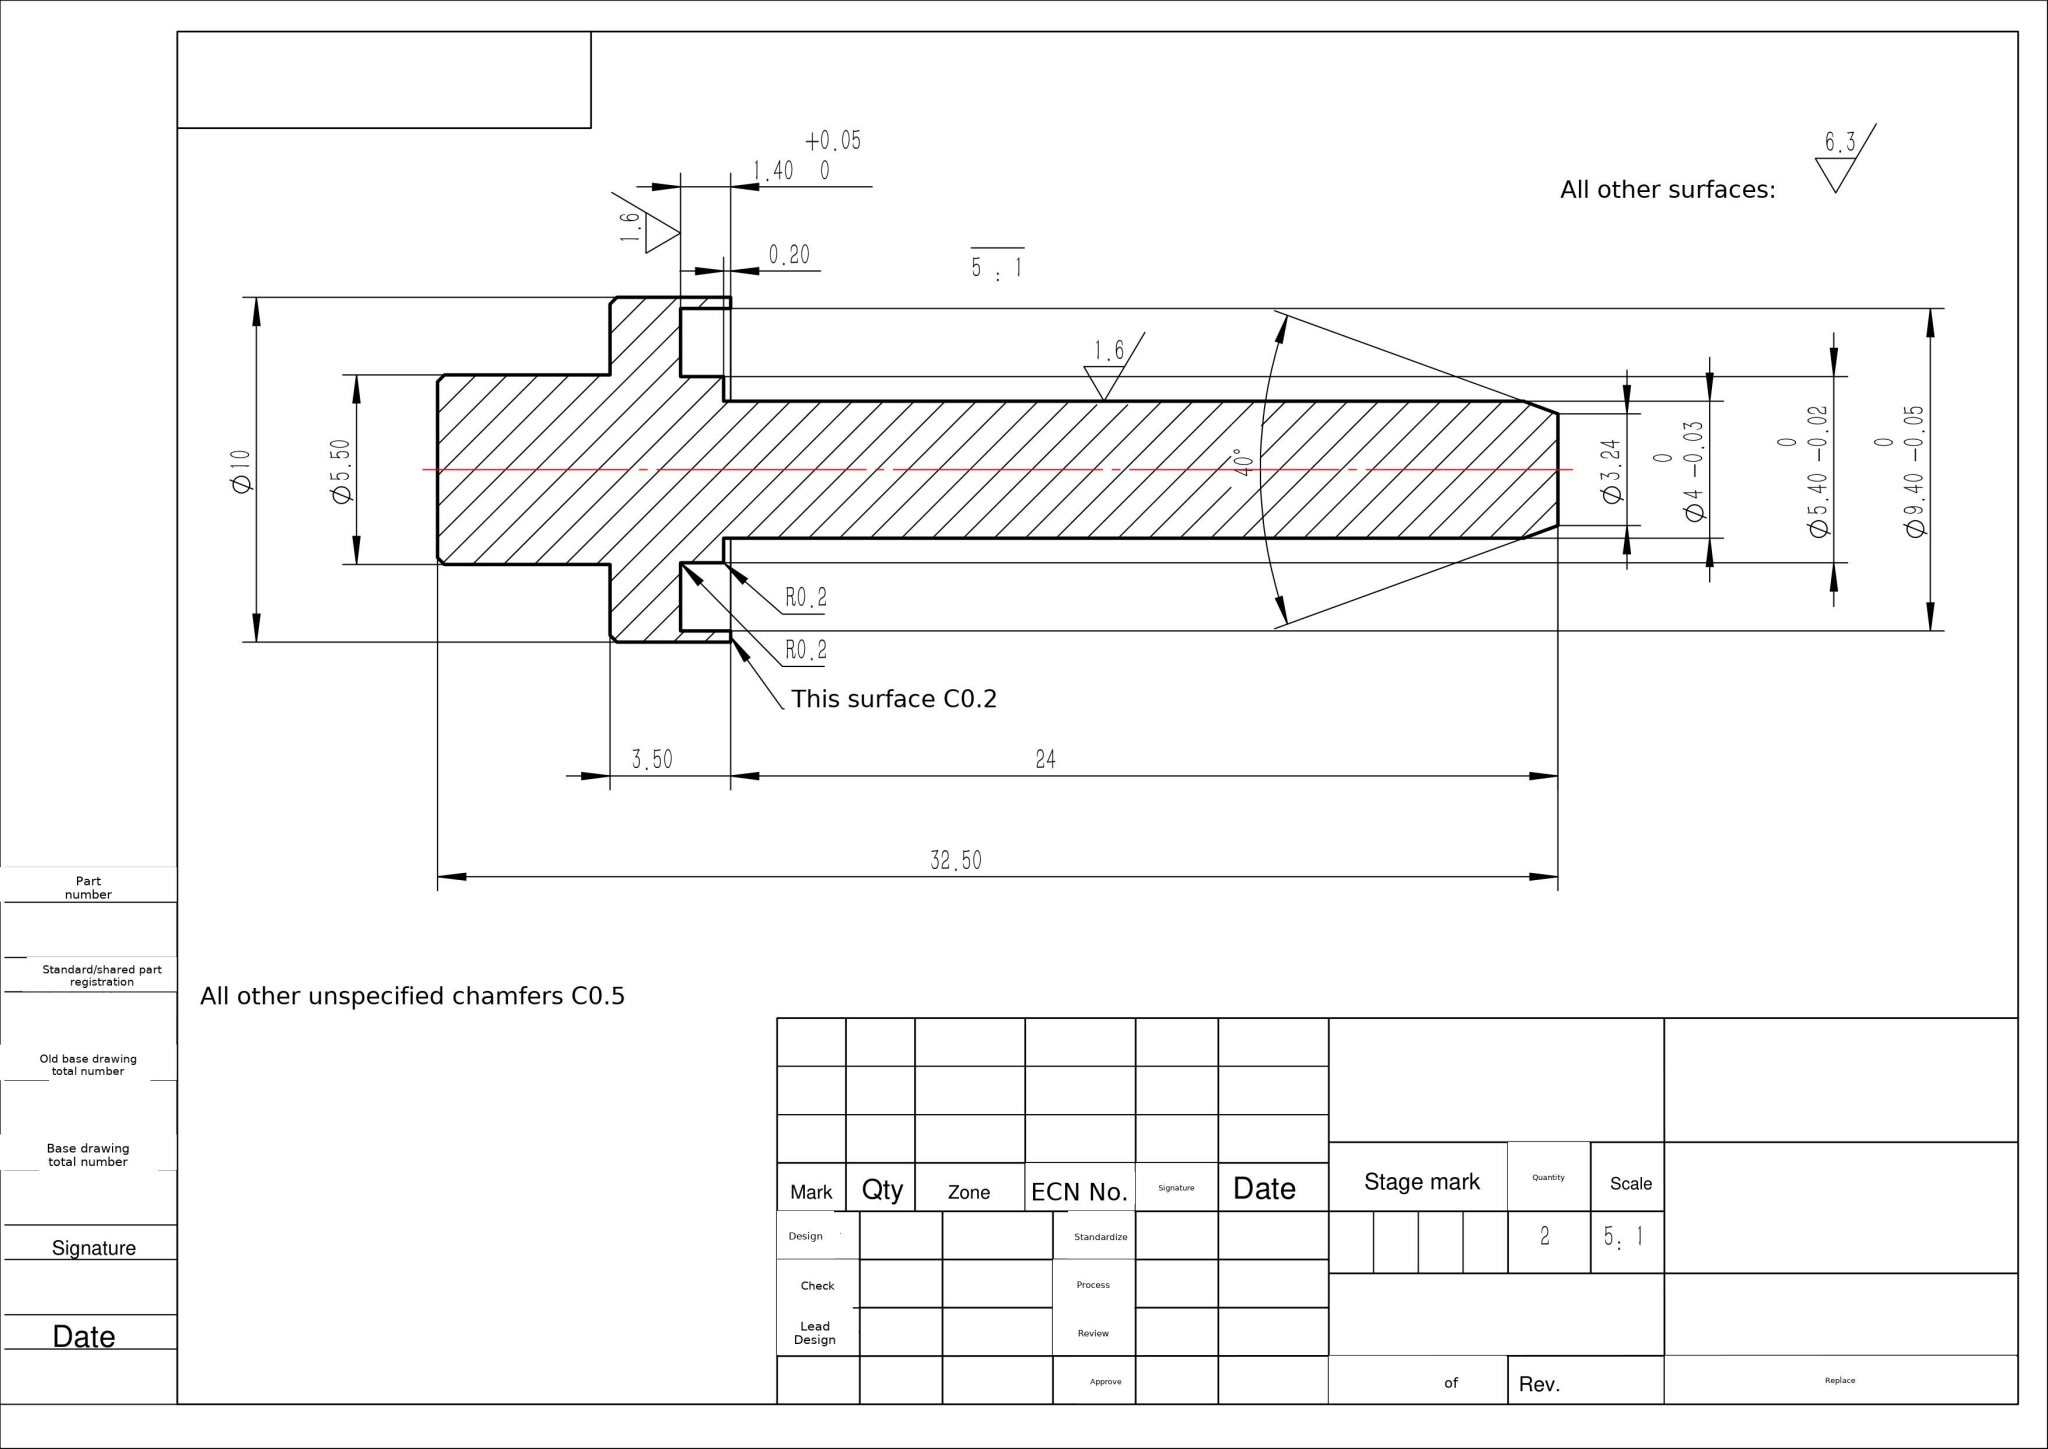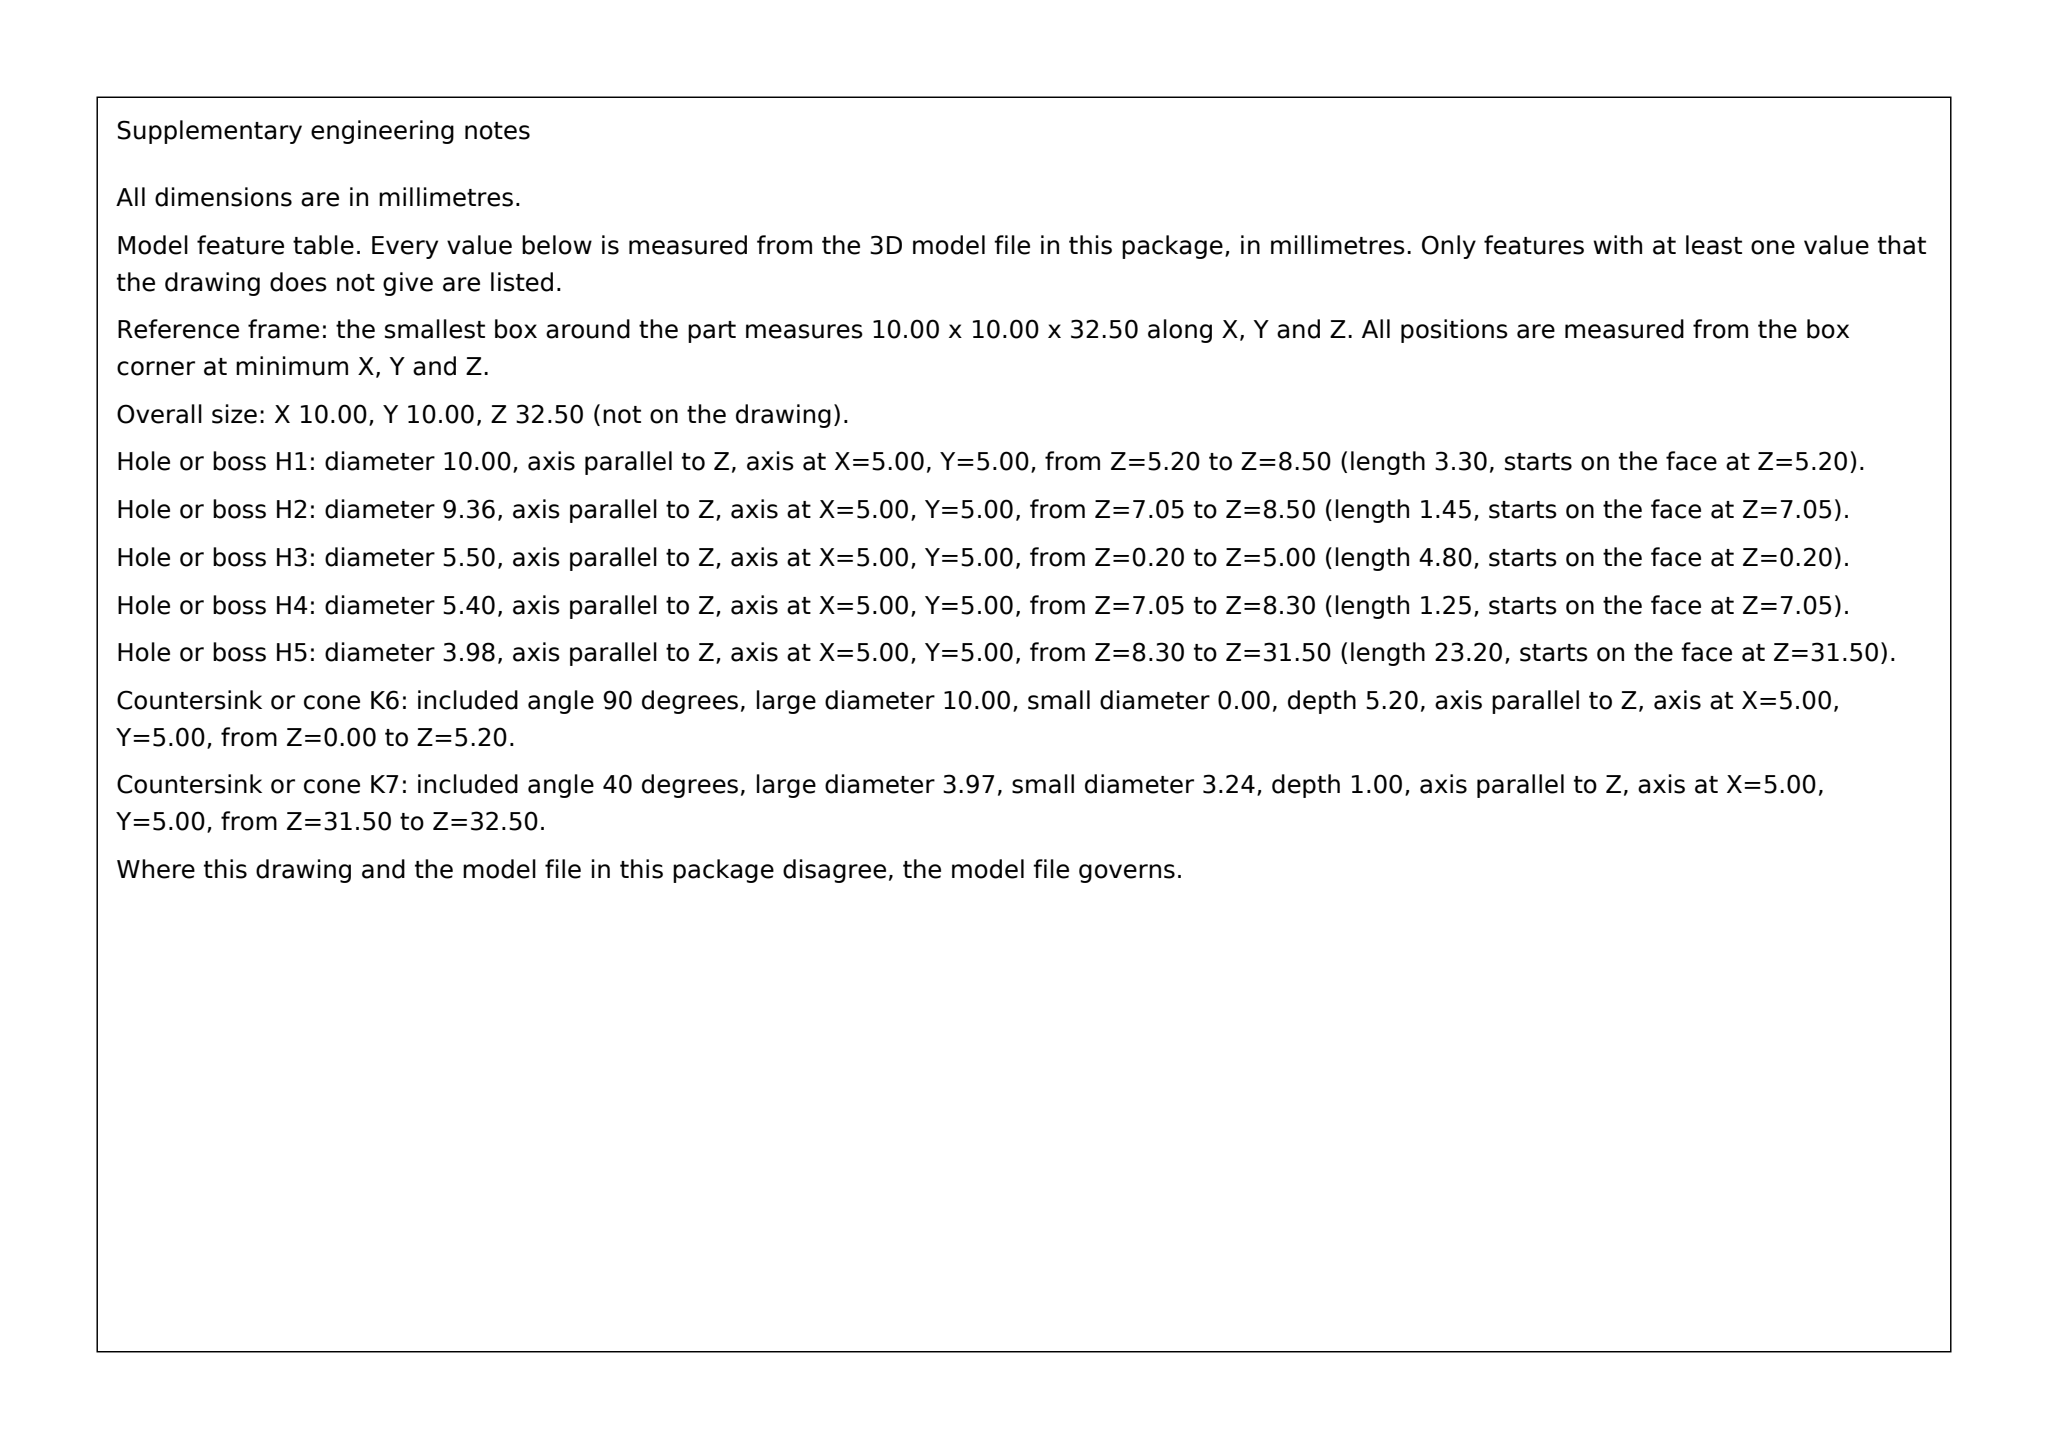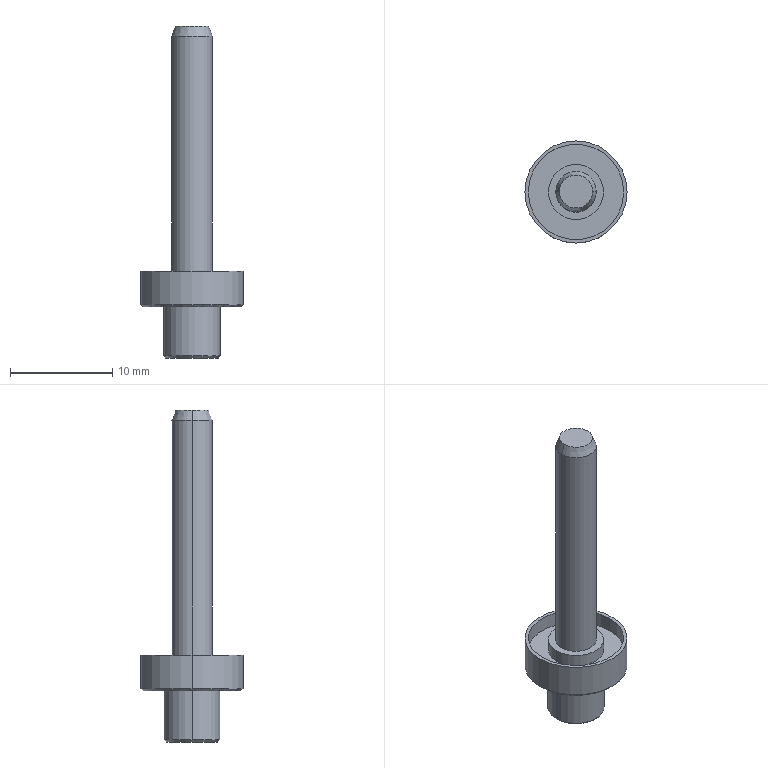Part | SolidWorks | mm | 1 solid | 22 faces | box 10 x 10 x 32.5 mm | volume 619 mm3 | cylinder 10 | cone 6 | plane 6 | commonest cylinder face diameters 3.97 x2 5.4 x2 9.35 x2 10 x2 5.5 x2
build123d program:
from build123d import *

# Parameters (mm, degrees)
CHAMFER1_SIZE  = 0.2
CHAMFER2_SIZE  = 1
CHAMFER2_SIZE2 = 0.364


with BuildPart() as part:
    # Sketch1 → Revolve1 (revolve)
    with BuildSketch(Plane(origin=(0, 0, 0), x_dir=(0, 0, -1), z_dir=(1, 0, 0)), mode=Mode.PRIVATE) as revolve1_sk:
        Polygon((32.5, 0), (32.5, 2.75), (27.5, 2.75), (27.5, 5), (24, 5), (24, 4.675), (25.45, 4.675), (25.45, 2.7), (24.2, 2.7), (24.2, 1.985), (0, 1.985), (0, 0), align=None)
    revolve(revolve1_sk.sketch.rotate(Axis((0, 0, 0), (0, 0, -1)), 90), axis=Axis((0, 0, 0), (0, 0, -1)))

    # Chamfer1
    chamfer1_edges = [part.edges().sort_by_distance(p)[0] for p in [
        (-5, 0, -27.5),
        (-2.75, 0, -32.5),
    ]]
    chamfer(chamfer1_edges, length=CHAMFER1_SIZE)

    # Chamfer2
    chamfer2_edges = [part.edges().sort_by_distance(p)[0] for p in [
        (-1.985, 0, 0),
    ]]
    chamfer2_side = [part.faces().sort_by_distance(p)[0] for p in [
        (-1.985, 0, -12.1),
    ]]
    chamfer(chamfer2_edges, length=CHAMFER2_SIZE, length2=CHAMFER2_SIZE2, reference=chamfer2_side[0])


solid = part.part
STEP:
#1=CARTESIAN_POINT('',(1.621,0.,-0.));
#2=VERTEX_POINT('',#1);
#3=CARTESIAN_POINT('',(-1.621,0.,-0.));
#4=VERTEX_POINT('',#3);
#5=CARTESIAN_POINT('',(0.,0.,0.));
#6=DIRECTION('',(0.,0.,1.));
#7=DIRECTION('',(-1.,0.,-0.));
#8=AXIS2_PLACEMENT_3D('',#5,#6,#7);
#9=CIRCLE('',#8,1.621);
#10=EDGE_CURVE('',#2,#4,#9,.T.);
#11=ORIENTED_EDGE('',*,*,#10,.F.);
#12=CARTESIAN_POINT('',(1.985,-0.,-1.));
#13=VERTEX_POINT('',#12);
#14=CARTESIAN_POINT('',(1.621,0.,0.));
#15=DIRECTION('',(0.342,0.,-0.9397));
#16=VECTOR('',#15,1000.);
#17=LINE('',#14,#16);
#18=EDGE_CURVE('',#2,#13,#17,.T.);
#19=ORIENTED_EDGE('',*,*,#18,.T.);
#20=CARTESIAN_POINT('',(-1.985,0.,-1.));
#21=VERTEX_POINT('',#20);
#22=CARTESIAN_POINT('',(0.,0.,-1.));
#23=DIRECTION('',(-0.,-0.,-1.));
#24=DIRECTION('',(-1.,0.,0.));
#25=AXIS2_PLACEMENT_3D('',#22,#23,#24);
#26=CIRCLE('',#25,1.985);
#27=EDGE_CURVE('',#21,#13,#26,.T.);
#28=ORIENTED_EDGE('',*,*,#27,.F.);
#29=CARTESIAN_POINT('',(-1.621,0.,-0.));
#30=DIRECTION('',(-0.342,0.,-0.9397));
#31=VECTOR('',#30,1000.);
#32=LINE('',#29,#31);
#33=EDGE_CURVE('',#4,#21,#32,.T.);
#34=ORIENTED_EDGE('',*,*,#33,.F.);
#35=EDGE_LOOP('',(#11,#19,#28,#34));
#36=FACE_OUTER_BOUND('',#35,.T.);
#37=CARTESIAN_POINT('',(0.,0.,0.));
#38=DIRECTION('',(-0.,-0.,-1.));
#39=DIRECTION('',(-1.,0.,-0.));
#40=AXIS2_PLACEMENT_3D('',#37,#38,#39);
#41=CONICAL_SURFACE('',#40,1.621,0.3491);
#42=ADVANCED_FACE('',(#36),#41,.T.);
#43=CARTESIAN_POINT('',(-2.55,0.,-32.5));
#44=VERTEX_POINT('',#43);
#45=CARTESIAN_POINT('',(2.55,0.,-32.5));
#46=VERTEX_POINT('',#45);
#47=CARTESIAN_POINT('',(0.,0.,-32.5));
#48=DIRECTION('',(-0.,-0.,-1.));
#49=DIRECTION('',(1.,-0.,0.));
#50=AXIS2_PLACEMENT_3D('',#47,#48,#49);
#51=CIRCLE('',#50,2.55);
#52=EDGE_CURVE('',#44,#46,#51,.T.);
#53=ORIENTED_EDGE('',*,*,#52,.F.);
#54=CARTESIAN_POINT('',(-2.75,0.,-32.3));
#55=VERTEX_POINT('',#54);
#56=CARTESIAN_POINT('',(-2.75,0.,-32.3));
#57=DIRECTION('',(-0.7071,0.,0.7071));
#58=VECTOR('',#57,1000.);
#59=LINE('',#56,#58);
#60=EDGE_CURVE('',#44,#55,#59,.T.);
#61=ORIENTED_EDGE('',*,*,#60,.T.);
#62=CARTESIAN_POINT('',(2.75,0.,-32.3));
#63=VERTEX_POINT('',#62);
#64=CARTESIAN_POINT('',(0.,0.,-32.3));
#65=DIRECTION('',(0.,0.,1.));
#66=DIRECTION('',(1.,-0.,0.));
#67=AXIS2_PLACEMENT_3D('',#64,#65,#66);
#68=CIRCLE('',#67,2.75);
#69=EDGE_CURVE('',#63,#55,#68,.T.);
#70=ORIENTED_EDGE('',*,*,#69,.F.);
#71=CARTESIAN_POINT('',(2.75,0.,-32.3));
#72=DIRECTION('',(0.7071,-0.,0.7071));
#73=VECTOR('',#72,1000.);
#74=LINE('',#71,#73);
#75=EDGE_CURVE('',#46,#63,#74,.T.);
#76=ORIENTED_EDGE('',*,*,#75,.F.);
#77=EDGE_LOOP('',(#53,#61,#70,#76));
#78=FACE_OUTER_BOUND('',#77,.T.);
#79=CARTESIAN_POINT('',(0.,0.,-32.3));
#80=DIRECTION('',(0.,0.,1.));
#81=DIRECTION('',(1.,-0.,0.));
#82=AXIS2_PLACEMENT_3D('',#79,#80,#81);
#83=CONICAL_SURFACE('',#82,2.75,0.7854);
#84=ADVANCED_FACE('',(#78),#83,.T.);
#85=CARTESIAN_POINT('',(-4.8,0.,-27.5));
#86=VERTEX_POINT('',#85);
#87=CARTESIAN_POINT('',(4.8,0.,-27.5));
#88=VERTEX_POINT('',#87);
#89=CARTESIAN_POINT('',(0.,0.,-27.5));
#90=DIRECTION('',(-0.,-0.,-1.));
#91=DIRECTION('',(1.,-0.,0.));
#92=AXIS2_PLACEMENT_3D('',#89,#90,#91);
#93=CIRCLE('',#92,4.8);
#94=EDGE_CURVE('',#86,#88,#93,.T.);
#95=ORIENTED_EDGE('',*,*,#94,.F.);
#96=CARTESIAN_POINT('',(-5.,0.,-27.3));
#97=VERTEX_POINT('',#96);
#98=CARTESIAN_POINT('',(-5.,0.,-27.3));
#99=DIRECTION('',(-0.7071,0.,0.7071));
#100=VECTOR('',#99,1000.);
#101=LINE('',#98,#100);
#102=EDGE_CURVE('',#86,#97,#101,.T.);
#103=ORIENTED_EDGE('',*,*,#102,.T.);
#104=CARTESIAN_POINT('',(5.,0.,-27.3));
#105=VERTEX_POINT('',#104);
#106=CARTESIAN_POINT('',(0.,0.,-27.3));
#107=DIRECTION('',(0.,0.,1.));
#108=DIRECTION('',(1.,-0.,0.));
#109=AXIS2_PLACEMENT_3D('',#106,#107,#108);
#110=CIRCLE('',#109,5.);
#111=EDGE_CURVE('',#105,#97,#110,.T.);
#112=ORIENTED_EDGE('',*,*,#111,.F.);
#113=CARTESIAN_POINT('',(5.,0.,-27.3));
#114=DIRECTION('',(0.7071,-0.,0.7071));
#115=VECTOR('',#114,1000.);
#116=LINE('',#113,#115);
#117=EDGE_CURVE('',#88,#105,#116,.T.);
#118=ORIENTED_EDGE('',*,*,#117,.F.);
#119=EDGE_LOOP('',(#95,#103,#112,#118));
#120=FACE_OUTER_BOUND('',#119,.T.);
#121=CARTESIAN_POINT('',(0.,0.,-27.3));
#122=DIRECTION('',(0.,0.,1.));
#123=DIRECTION('',(1.,-0.,0.));
#124=AXIS2_PLACEMENT_3D('',#121,#122,#123);
#125=CONICAL_SURFACE('',#124,5.,0.7854);
#126=ADVANCED_FACE('',(#120),#125,.T.);
#127=CARTESIAN_POINT('',(1.985,0.,-24.2));
#128=VERTEX_POINT('',#127);
#129=CARTESIAN_POINT('',(-1.985,0.,-24.2));
#130=VERTEX_POINT('',#129);
#131=CARTESIAN_POINT('',(0.,0.,-24.2));
#132=DIRECTION('',(0.,0.,1.));
#133=DIRECTION('',(1.,-0.,0.));
#134=AXIS2_PLACEMENT_3D('',#131,#132,#133);
#135=CIRCLE('',#134,1.985);
#136=EDGE_CURVE('',#128,#130,#135,.T.);
#137=ORIENTED_EDGE('',*,*,#136,.T.);
#138=CARTESIAN_POINT('',(-1.985,0.,-0.));
#139=DIRECTION('',(0.,0.,1.));
#140=VECTOR('',#139,1000.);
#141=LINE('',#138,#140);
#142=EDGE_CURVE('',#130,#21,#141,.T.);
#143=ORIENTED_EDGE('',*,*,#142,.T.);
#144=ORIENTED_EDGE('',*,*,#27,.T.);
#145=CARTESIAN_POINT('',(1.985,-0.,0.));
#146=DIRECTION('',(0.,0.,1.));
#147=VECTOR('',#146,1000.);
#148=LINE('',#145,#147);
#149=EDGE_CURVE('',#128,#13,#148,.T.);
#150=ORIENTED_EDGE('',*,*,#149,.F.);
#151=EDGE_LOOP('',(#137,#143,#144,#150));
#152=FACE_OUTER_BOUND('',#151,.T.);
#153=CARTESIAN_POINT('',(0.,0.,0.));
#154=DIRECTION('',(0.,0.,1.));
#155=DIRECTION('',(1.,-0.,0.));
#156=AXIS2_PLACEMENT_3D('',#153,#154,#155);
#157=CYLINDRICAL_SURFACE('',#156,1.985);
#158=ADVANCED_FACE('',(#152),#157,.T.);
#159=CARTESIAN_POINT('',(2.7,0.,-25.45));
#160=VERTEX_POINT('',#159);
#161=CARTESIAN_POINT('',(-2.7,0.,-25.45));
#162=VERTEX_POINT('',#161);
#163=CARTESIAN_POINT('',(0.,0.,-25.45));
#164=DIRECTION('',(0.,0.,1.));
#165=DIRECTION('',(1.,-0.,0.));
#166=AXIS2_PLACEMENT_3D('',#163,#164,#165);
#167=CIRCLE('',#166,2.7);
#168=EDGE_CURVE('',#160,#162,#167,.T.);
#169=ORIENTED_EDGE('',*,*,#168,.T.);
#170=CARTESIAN_POINT('',(-2.7,0.,-24.2));
#171=VERTEX_POINT('',#170);
#172=CARTESIAN_POINT('',(-2.7,0.,-0.));
#173=DIRECTION('',(0.,0.,1.));
#174=VECTOR('',#173,1000.);
#175=LINE('',#172,#174);
#176=EDGE_CURVE('',#162,#171,#175,.T.);
#177=ORIENTED_EDGE('',*,*,#176,.T.);
#178=CARTESIAN_POINT('',(2.7,0.,-24.2));
#179=VERTEX_POINT('',#178);
#180=CARTESIAN_POINT('',(0.,0.,-24.2));
#181=DIRECTION('',(0.,0.,1.));
#182=DIRECTION('',(1.,-0.,0.));
#183=AXIS2_PLACEMENT_3D('',#180,#181,#182);
#184=CIRCLE('',#183,2.7);
#185=EDGE_CURVE('',#179,#171,#184,.T.);
#186=ORIENTED_EDGE('',*,*,#185,.F.);
#187=CARTESIAN_POINT('',(2.7,-0.,0.));
#188=DIRECTION('',(0.,0.,1.));
#189=VECTOR('',#188,1000.);
#190=LINE('',#187,#189);
#191=EDGE_CURVE('',#160,#179,#190,.T.);
#192=ORIENTED_EDGE('',*,*,#191,.F.);
#193=EDGE_LOOP('',(#169,#177,#186,#192));
#194=FACE_OUTER_BOUND('',#193,.T.);
#195=CARTESIAN_POINT('',(0.,0.,0.));
#196=DIRECTION('',(0.,0.,1.));
#197=DIRECTION('',(1.,-0.,0.));
#198=AXIS2_PLACEMENT_3D('',#195,#196,#197);
#199=CYLINDRICAL_SURFACE('',#198,2.7);
#200=ADVANCED_FACE('',(#194),#199,.T.);
#201=CARTESIAN_POINT('',(-4.675,0.,-25.45));
#202=VERTEX_POINT('',#201);
#203=CARTESIAN_POINT('',(4.675,0.,-25.45));
#204=VERTEX_POINT('',#203);
#205=CARTESIAN_POINT('',(0.,0.,-25.45));
#206=DIRECTION('',(0.,0.,1.));
#207=DIRECTION('',(1.,-0.,0.));
#208=AXIS2_PLACEMENT_3D('',#205,#206,#207);
#209=CIRCLE('',#208,4.675);
#210=EDGE_CURVE('',#202,#204,#209,.T.);
#211=ORIENTED_EDGE('',*,*,#210,.F.);
#212=CARTESIAN_POINT('',(-4.675,0.,-24.));
#213=VERTEX_POINT('',#212);
#214=CARTESIAN_POINT('',(-4.675,0.,-0.));
#215=DIRECTION('',(0.,0.,1.));
#216=VECTOR('',#215,1000.);
#217=LINE('',#214,#216);
#218=EDGE_CURVE('',#202,#213,#217,.T.);
#219=ORIENTED_EDGE('',*,*,#218,.T.);
#220=CARTESIAN_POINT('',(4.675,0.,-24.));
#221=VERTEX_POINT('',#220);
#222=CARTESIAN_POINT('',(0.,0.,-24.));
#223=DIRECTION('',(0.,0.,1.));
#224=DIRECTION('',(1.,-0.,0.));
#225=AXIS2_PLACEMENT_3D('',#222,#223,#224);
#226=CIRCLE('',#225,4.675);
#227=EDGE_CURVE('',#213,#221,#226,.T.);
#228=ORIENTED_EDGE('',*,*,#227,.T.);
#229=CARTESIAN_POINT('',(4.675,-0.,0.));
#230=DIRECTION('',(0.,0.,1.));
#231=VECTOR('',#230,1000.);
#232=LINE('',#229,#231);
#233=EDGE_CURVE('',#204,#221,#232,.T.);
#234=ORIENTED_EDGE('',*,*,#233,.F.);
#235=EDGE_LOOP('',(#211,#219,#228,#234));
#236=FACE_OUTER_BOUND('',#235,.T.);
#237=CARTESIAN_POINT('',(0.,0.,0.));
#238=DIRECTION('',(0.,0.,1.));
#239=DIRECTION('',(1.,-0.,0.));
#240=AXIS2_PLACEMENT_3D('',#237,#238,#239);
#241=CYLINDRICAL_SURFACE('',#240,4.675);
#242=ADVANCED_FACE('',(#236),#241,.F.);
#243=ORIENTED_EDGE('',*,*,#111,.T.);
#244=CARTESIAN_POINT('',(-5.,0.,-24.));
#245=VERTEX_POINT('',#244);
#246=CARTESIAN_POINT('',(-5.,0.,-0.));
#247=DIRECTION('',(0.,0.,1.));
#248=VECTOR('',#247,1000.);
#249=LINE('',#246,#248);
#250=EDGE_CURVE('',#97,#245,#249,.T.);
#251=ORIENTED_EDGE('',*,*,#250,.T.);
#252=CARTESIAN_POINT('',(5.,0.,-24.));
#253=VERTEX_POINT('',#252);
#254=CARTESIAN_POINT('',(0.,0.,-24.));
#255=DIRECTION('',(0.,0.,1.));
#256=DIRECTION('',(1.,-0.,0.));
#257=AXIS2_PLACEMENT_3D('',#254,#255,#256);
#258=CIRCLE('',#257,5.);
#259=EDGE_CURVE('',#253,#245,#258,.T.);
#260=ORIENTED_EDGE('',*,*,#259,.F.);
#261=CARTESIAN_POINT('',(5.,-0.,0.));
#262=DIRECTION('',(0.,0.,1.));
#263=VECTOR('',#262,1000.);
#264=LINE('',#261,#263);
#265=EDGE_CURVE('',#105,#253,#264,.T.);
#266=ORIENTED_EDGE('',*,*,#265,.F.);
#267=EDGE_LOOP('',(#243,#251,#260,#266));
#268=FACE_OUTER_BOUND('',#267,.T.);
#269=CARTESIAN_POINT('',(0.,0.,0.));
#270=DIRECTION('',(0.,0.,1.));
#271=DIRECTION('',(1.,-0.,0.));
#272=AXIS2_PLACEMENT_3D('',#269,#270,#271);
#273=CYLINDRICAL_SURFACE('',#272,5.);
#274=ADVANCED_FACE('',(#268),#273,.T.);
#275=ORIENTED_EDGE('',*,*,#69,.T.);
#276=CARTESIAN_POINT('',(-2.75,0.,-27.5));
#277=VERTEX_POINT('',#276);
#278=CARTESIAN_POINT('',(-2.75,0.,-0.));
#279=DIRECTION('',(0.,0.,1.));
#280=VECTOR('',#279,1000.);
#281=LINE('',#278,#280);
#282=EDGE_CURVE('',#55,#277,#281,.T.);
#283=ORIENTED_EDGE('',*,*,#282,.T.);
#284=CARTESIAN_POINT('',(2.75,0.,-27.5));
#285=VERTEX_POINT('',#284);
#286=CARTESIAN_POINT('',(0.,0.,-27.5));
#287=DIRECTION('',(0.,0.,1.));
#288=DIRECTION('',(1.,-0.,0.));
#289=AXIS2_PLACEMENT_3D('',#286,#287,#288);
#290=CIRCLE('',#289,2.75);
#291=EDGE_CURVE('',#285,#277,#290,.T.);
#292=ORIENTED_EDGE('',*,*,#291,.F.);
#293=CARTESIAN_POINT('',(2.75,-0.,0.));
#294=DIRECTION('',(0.,0.,1.));
#295=VECTOR('',#294,1000.);
#296=LINE('',#293,#295);
#297=EDGE_CURVE('',#63,#285,#296,.T.);
#298=ORIENTED_EDGE('',*,*,#297,.F.);
#299=EDGE_LOOP('',(#275,#283,#292,#298));
#300=FACE_OUTER_BOUND('',#299,.T.);
#301=CARTESIAN_POINT('',(0.,0.,0.));
#302=DIRECTION('',(0.,0.,1.));
#303=DIRECTION('',(1.,-0.,0.));
#304=AXIS2_PLACEMENT_3D('',#301,#302,#303);
#305=CYLINDRICAL_SURFACE('',#304,2.75);
#306=ADVANCED_FACE('',(#300),#305,.T.);
#307=CARTESIAN_POINT('',(0.,0.,-32.5));
#308=DIRECTION('',(-0.,-0.,-1.));
#309=DIRECTION('',(1.,-0.,0.));
#310=AXIS2_PLACEMENT_3D('',#307,#308,#309);
#311=CIRCLE('',#310,2.55);
#312=EDGE_CURVE('',#46,#44,#311,.T.);
#313=ORIENTED_EDGE('',*,*,#312,.T.);
#314=ORIENTED_EDGE('',*,*,#52,.T.);
#315=EDGE_LOOP('',(#313,#314));
#316=FACE_OUTER_BOUND('',#315,.T.);
#317=CARTESIAN_POINT('',(0.,0.,-32.5));
#318=DIRECTION('',(-0.,0.,1.));
#319=DIRECTION('',(1.,-0.,0.));
#320=AXIS2_PLACEMENT_3D('',#317,#318,#319);
#321=PLANE('',#320);
#322=ADVANCED_FACE('',(#316),#321,.F.);
#323=ORIENTED_EDGE('',*,*,#282,.F.);
#324=CARTESIAN_POINT('',(0.,0.,-32.3));
#325=DIRECTION('',(0.,0.,1.));
#326=DIRECTION('',(1.,-0.,0.));
#327=AXIS2_PLACEMENT_3D('',#324,#325,#326);
#328=CIRCLE('',#327,2.75);
#329=EDGE_CURVE('',#55,#63,#328,.T.);
#330=ORIENTED_EDGE('',*,*,#329,.T.);
#331=ORIENTED_EDGE('',*,*,#297,.T.);
#332=CARTESIAN_POINT('',(0.,0.,-27.5));
#333=DIRECTION('',(0.,0.,1.));
#334=DIRECTION('',(1.,-0.,0.));
#335=AXIS2_PLACEMENT_3D('',#332,#333,#334);
#336=CIRCLE('',#335,2.75);
#337=EDGE_CURVE('',#277,#285,#336,.T.);
#338=ORIENTED_EDGE('',*,*,#337,.F.);
#339=EDGE_LOOP('',(#323,#330,#331,#338));
#340=FACE_OUTER_BOUND('',#339,.T.);
#341=CARTESIAN_POINT('',(0.,0.,0.));
#342=DIRECTION('',(0.,0.,1.));
#343=DIRECTION('',(1.,-0.,0.));
#344=AXIS2_PLACEMENT_3D('',#341,#342,#343);
#345=CYLINDRICAL_SURFACE('',#344,2.75);
#346=ADVANCED_FACE('',(#340),#345,.T.);
#347=CARTESIAN_POINT('',(0.,0.,-27.5));
#348=DIRECTION('',(-0.,-0.,-1.));
#349=DIRECTION('',(1.,-0.,0.));
#350=AXIS2_PLACEMENT_3D('',#347,#348,#349);
#351=CIRCLE('',#350,4.8);
#352=EDGE_CURVE('',#88,#86,#351,.T.);
#353=ORIENTED_EDGE('',*,*,#352,.T.);
#354=ORIENTED_EDGE('',*,*,#94,.T.);
#355=EDGE_LOOP('',(#353,#354));
#356=FACE_OUTER_BOUND('',#355,.T.);
#357=ORIENTED_EDGE('',*,*,#291,.T.);
#358=ORIENTED_EDGE('',*,*,#337,.T.);
#359=EDGE_LOOP('',(#357,#358));
#360=FACE_BOUND('',#359,.T.);
#361=CARTESIAN_POINT('',(0.,2.75,-27.5));
#362=DIRECTION('',(-0.,0.,1.));
#363=DIRECTION('',(1.,-0.,0.));
#364=AXIS2_PLACEMENT_3D('',#361,#362,#363);
#365=PLANE('',#364);
#366=ADVANCED_FACE('',(#356,#360),#365,.F.);
#367=ORIENTED_EDGE('',*,*,#250,.F.);
#368=CARTESIAN_POINT('',(0.,0.,-27.3));
#369=DIRECTION('',(0.,0.,1.));
#370=DIRECTION('',(1.,-0.,0.));
#371=AXIS2_PLACEMENT_3D('',#368,#369,#370);
#372=CIRCLE('',#371,5.);
#373=EDGE_CURVE('',#97,#105,#372,.T.);
#374=ORIENTED_EDGE('',*,*,#373,.T.);
#375=ORIENTED_EDGE('',*,*,#265,.T.);
#376=CARTESIAN_POINT('',(0.,0.,-24.));
#377=DIRECTION('',(0.,0.,1.));
#378=DIRECTION('',(1.,-0.,0.));
#379=AXIS2_PLACEMENT_3D('',#376,#377,#378);
#380=CIRCLE('',#379,5.);
#381=EDGE_CURVE('',#245,#253,#380,.T.);
#382=ORIENTED_EDGE('',*,*,#381,.F.);
#383=EDGE_LOOP('',(#367,#374,#375,#382));
#384=FACE_OUTER_BOUND('',#383,.T.);
#385=CARTESIAN_POINT('',(0.,0.,0.));
#386=DIRECTION('',(0.,0.,1.));
#387=DIRECTION('',(1.,-0.,0.));
#388=AXIS2_PLACEMENT_3D('',#385,#386,#387);
#389=CYLINDRICAL_SURFACE('',#388,5.);
#390=ADVANCED_FACE('',(#384),#389,.T.);
#391=CARTESIAN_POINT('',(0.,0.,-24.));
#392=DIRECTION('',(0.,0.,1.));
#393=DIRECTION('',(1.,-0.,0.));
#394=AXIS2_PLACEMENT_3D('',#391,#392,#393);
#395=CIRCLE('',#394,4.675);
#396=EDGE_CURVE('',#221,#213,#395,.T.);
#397=ORIENTED_EDGE('',*,*,#396,.F.);
#398=ORIENTED_EDGE('',*,*,#227,.F.);
#399=EDGE_LOOP('',(#397,#398));
#400=FACE_BOUND('',#399,.T.);
#401=ORIENTED_EDGE('',*,*,#259,.T.);
#402=ORIENTED_EDGE('',*,*,#381,.T.);
#403=EDGE_LOOP('',(#401,#402));
#404=FACE_OUTER_BOUND('',#403,.T.);
#405=CARTESIAN_POINT('',(0.,5.,-24.));
#406=DIRECTION('',(0.,-0.,-1.));
#407=DIRECTION('',(-1.,0.,-0.));
#408=AXIS2_PLACEMENT_3D('',#405,#406,#407);
#409=PLANE('',#408);
#410=ADVANCED_FACE('',(#400,#404),#409,.F.);
#411=ORIENTED_EDGE('',*,*,#218,.F.);
#412=CARTESIAN_POINT('',(0.,0.,-25.45));
#413=DIRECTION('',(0.,0.,1.));
#414=DIRECTION('',(1.,-0.,0.));
#415=AXIS2_PLACEMENT_3D('',#412,#413,#414);
#416=CIRCLE('',#415,4.675);
#417=EDGE_CURVE('',#204,#202,#416,.T.);
#418=ORIENTED_EDGE('',*,*,#417,.F.);
#419=ORIENTED_EDGE('',*,*,#233,.T.);
#420=ORIENTED_EDGE('',*,*,#396,.T.);
#421=EDGE_LOOP('',(#411,#418,#419,#420));
#422=FACE_OUTER_BOUND('',#421,.T.);
#423=CARTESIAN_POINT('',(0.,0.,0.));
#424=DIRECTION('',(0.,0.,1.));
#425=DIRECTION('',(1.,-0.,0.));
#426=AXIS2_PLACEMENT_3D('',#423,#424,#425);
#427=CYLINDRICAL_SURFACE('',#426,4.675);
#428=ADVANCED_FACE('',(#422),#427,.F.);
#429=ORIENTED_EDGE('',*,*,#168,.F.);
#430=CARTESIAN_POINT('',(0.,0.,-25.45));
#431=DIRECTION('',(0.,0.,1.));
#432=DIRECTION('',(1.,-0.,0.));
#433=AXIS2_PLACEMENT_3D('',#430,#431,#432);
#434=CIRCLE('',#433,2.7);
#435=EDGE_CURVE('',#162,#160,#434,.T.);
#436=ORIENTED_EDGE('',*,*,#435,.F.);
#437=EDGE_LOOP('',(#429,#436));
#438=FACE_BOUND('',#437,.T.);
#439=ORIENTED_EDGE('',*,*,#417,.T.);
#440=ORIENTED_EDGE('',*,*,#210,.T.);
#441=EDGE_LOOP('',(#439,#440));
#442=FACE_OUTER_BOUND('',#441,.T.);
#443=CARTESIAN_POINT('',(0.,4.675,-25.45));
#444=DIRECTION('',(0.,-0.,-1.));
#445=DIRECTION('',(-1.,0.,-0.));
#446=AXIS2_PLACEMENT_3D('',#443,#444,#445);
#447=PLANE('',#446);
#448=ADVANCED_FACE('',(#438,#442),#447,.F.);
#449=ORIENTED_EDGE('',*,*,#176,.F.);
#450=ORIENTED_EDGE('',*,*,#435,.T.);
#451=ORIENTED_EDGE('',*,*,#191,.T.);
#452=CARTESIAN_POINT('',(0.,0.,-24.2));
#453=DIRECTION('',(0.,0.,1.));
#454=DIRECTION('',(1.,-0.,0.));
#455=AXIS2_PLACEMENT_3D('',#452,#453,#454);
#456=CIRCLE('',#455,2.7);
#457=EDGE_CURVE('',#171,#179,#456,.T.);
#458=ORIENTED_EDGE('',*,*,#457,.F.);
#459=EDGE_LOOP('',(#449,#450,#451,#458));
#460=FACE_OUTER_BOUND('',#459,.T.);
#461=CARTESIAN_POINT('',(0.,0.,0.));
#462=DIRECTION('',(0.,0.,1.));
#463=DIRECTION('',(1.,-0.,0.));
#464=AXIS2_PLACEMENT_3D('',#461,#462,#463);
#465=CYLINDRICAL_SURFACE('',#464,2.7);
#466=ADVANCED_FACE('',(#460),#465,.T.);
#467=ORIENTED_EDGE('',*,*,#136,.F.);
#468=CARTESIAN_POINT('',(0.,0.,-24.2));
#469=DIRECTION('',(0.,0.,1.));
#470=DIRECTION('',(1.,-0.,0.));
#471=AXIS2_PLACEMENT_3D('',#468,#469,#470);
#472=CIRCLE('',#471,1.985);
#473=EDGE_CURVE('',#130,#128,#472,.T.);
#474=ORIENTED_EDGE('',*,*,#473,.F.);
#475=EDGE_LOOP('',(#467,#474));
#476=FACE_BOUND('',#475,.T.);
#477=ORIENTED_EDGE('',*,*,#185,.T.);
#478=ORIENTED_EDGE('',*,*,#457,.T.);
#479=EDGE_LOOP('',(#477,#478));
#480=FACE_OUTER_BOUND('',#479,.T.);
#481=CARTESIAN_POINT('',(0.,2.7,-24.2));
#482=DIRECTION('',(0.,-0.,-1.));
#483=DIRECTION('',(-1.,0.,-0.));
#484=AXIS2_PLACEMENT_3D('',#481,#482,#483);
#485=PLANE('',#484);
#486=ADVANCED_FACE('',(#476,#480),#485,.F.);
#487=ORIENTED_EDGE('',*,*,#142,.F.);
#488=ORIENTED_EDGE('',*,*,#473,.T.);
#489=ORIENTED_EDGE('',*,*,#149,.T.);
#490=CARTESIAN_POINT('',(0.,0.,-1.));
#491=DIRECTION('',(-0.,-0.,-1.));
#492=DIRECTION('',(-1.,0.,0.));
#493=AXIS2_PLACEMENT_3D('',#490,#491,#492);
#494=CIRCLE('',#493,1.985);
#495=EDGE_CURVE('',#13,#21,#494,.T.);
#496=ORIENTED_EDGE('',*,*,#495,.T.);
#497=EDGE_LOOP('',(#487,#488,#489,#496));
#498=FACE_OUTER_BOUND('',#497,.T.);
#499=CARTESIAN_POINT('',(0.,0.,0.));
#500=DIRECTION('',(0.,0.,1.));
#501=DIRECTION('',(1.,-0.,0.));
#502=AXIS2_PLACEMENT_3D('',#499,#500,#501);
#503=CYLINDRICAL_SURFACE('',#502,1.985);
#504=ADVANCED_FACE('',(#498),#503,.T.);
#505=CARTESIAN_POINT('',(0.,0.,0.));
#506=DIRECTION('',(0.,0.,1.));
#507=DIRECTION('',(-1.,0.,-0.));
#508=AXIS2_PLACEMENT_3D('',#505,#506,#507);
#509=CIRCLE('',#508,1.621);
#510=EDGE_CURVE('',#4,#2,#509,.T.);
#511=ORIENTED_EDGE('',*,*,#510,.T.);
#512=ORIENTED_EDGE('',*,*,#10,.T.);
#513=EDGE_LOOP('',(#511,#512));
#514=FACE_OUTER_BOUND('',#513,.T.);
#515=CARTESIAN_POINT('',(0.,1.985,0.));
#516=DIRECTION('',(0.,-0.,-1.));
#517=DIRECTION('',(-1.,0.,-0.));
#518=AXIS2_PLACEMENT_3D('',#515,#516,#517);
#519=PLANE('',#518);
#520=ADVANCED_FACE('',(#514),#519,.F.);
#521=ORIENTED_EDGE('',*,*,#102,.F.);
#522=ORIENTED_EDGE('',*,*,#352,.F.);
#523=ORIENTED_EDGE('',*,*,#117,.T.);
#524=ORIENTED_EDGE('',*,*,#373,.F.);
#525=EDGE_LOOP('',(#521,#522,#523,#524));
#526=FACE_OUTER_BOUND('',#525,.T.);
#527=CARTESIAN_POINT('',(0.,0.,-27.3));
#528=DIRECTION('',(0.,0.,1.));
#529=DIRECTION('',(1.,-0.,0.));
#530=AXIS2_PLACEMENT_3D('',#527,#528,#529);
#531=CONICAL_SURFACE('',#530,5.,0.7854);
#532=ADVANCED_FACE('',(#526),#531,.T.);
#533=ORIENTED_EDGE('',*,*,#60,.F.);
#534=ORIENTED_EDGE('',*,*,#312,.F.);
#535=ORIENTED_EDGE('',*,*,#75,.T.);
#536=ORIENTED_EDGE('',*,*,#329,.F.);
#537=EDGE_LOOP('',(#533,#534,#535,#536));
#538=FACE_OUTER_BOUND('',#537,.T.);
#539=CARTESIAN_POINT('',(0.,0.,-32.3));
#540=DIRECTION('',(0.,0.,1.));
#541=DIRECTION('',(1.,-0.,0.));
#542=AXIS2_PLACEMENT_3D('',#539,#540,#541);
#543=CONICAL_SURFACE('',#542,2.75,0.7854);
#544=ADVANCED_FACE('',(#538),#543,.T.);
#545=ORIENTED_EDGE('',*,*,#18,.F.);
#546=ORIENTED_EDGE('',*,*,#510,.F.);
#547=ORIENTED_EDGE('',*,*,#33,.T.);
#548=ORIENTED_EDGE('',*,*,#495,.F.);
#549=EDGE_LOOP('',(#545,#546,#547,#548));
#550=FACE_OUTER_BOUND('',#549,.T.);
#551=CARTESIAN_POINT('',(0.,0.,0.));
#552=DIRECTION('',(-0.,-0.,-1.));
#553=DIRECTION('',(-1.,0.,-0.));
#554=AXIS2_PLACEMENT_3D('',#551,#552,#553);
#555=CONICAL_SURFACE('',#554,1.621,0.3491);
#556=ADVANCED_FACE('',(#550),#555,.T.);
#557=CLOSED_SHELL('',(#42,#84,#126,#158,#200,#242,#274,#306,#322,#346,#366,#390,#410,#428,#448,#466,#486,#504,#520,#532,#544,#556));
#558=MANIFOLD_SOLID_BREP('',#557);
#559=CARTESIAN_POINT('',(0.,0.,0.));
#560=DIRECTION('',(0.,0.,1.));
#561=DIRECTION('',(1.,0.,0.));
#562=AXIS2_PLACEMENT_3D('',#559,#560,#561);
#563=(LENGTH_UNIT()NAMED_UNIT(*)SI_UNIT(.MILLI.,.METRE.));
#564=UNCERTAINTY_MEASURE_WITH_UNIT(LENGTH_MEASURE(0.00001),#563,'','');
#565=(NAMED_UNIT(*)PLANE_ANGLE_UNIT()SI_UNIT($,.RADIAN.));
#566=(NAMED_UNIT(*)SI_UNIT($,.STERADIAN.)SOLID_ANGLE_UNIT());
#567=(GEOMETRIC_REPRESENTATION_CONTEXT(3)GLOBAL_UNCERTAINTY_ASSIGNED_CONTEXT((#564))GLOBAL_UNIT_ASSIGNED_CONTEXT((#563,#565,#566))REPRESENTATION_CONTEXT('',''));
#568=ADVANCED_BREP_SHAPE_REPRESENTATION('',(#558,#562),#567);